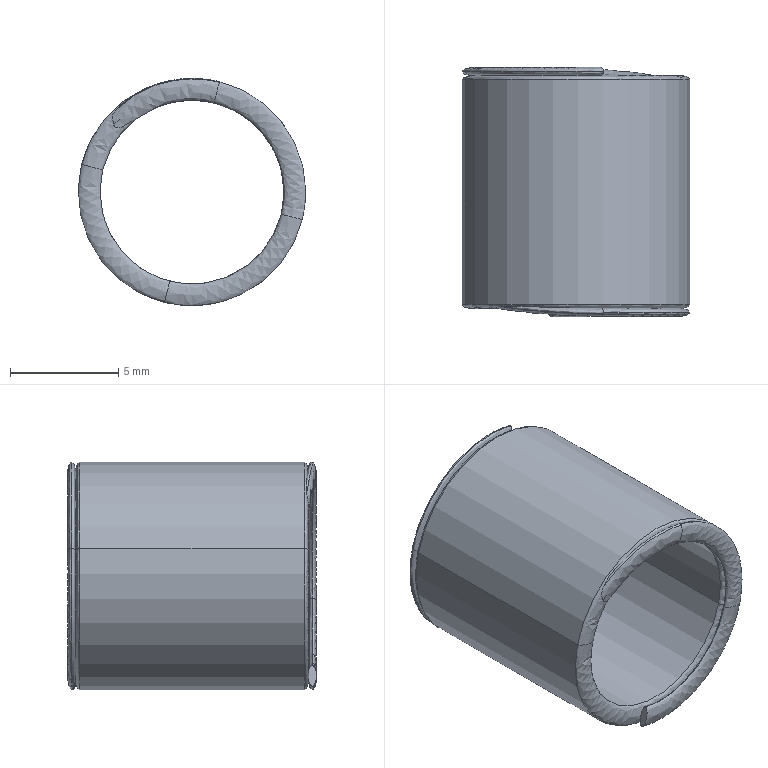Component | SolidWorks | 04LowerMaterialReceivingSwingAngleAssembly(3920)-1_RoundWireSpringYNWL-D8.5-L30-5 | 1 solid | 30 faces | volume 330 mm3 | spline 22 | cylinder 4 | plane 4 | commonest cylinder face diameters 10.5 x2 8.5 x2